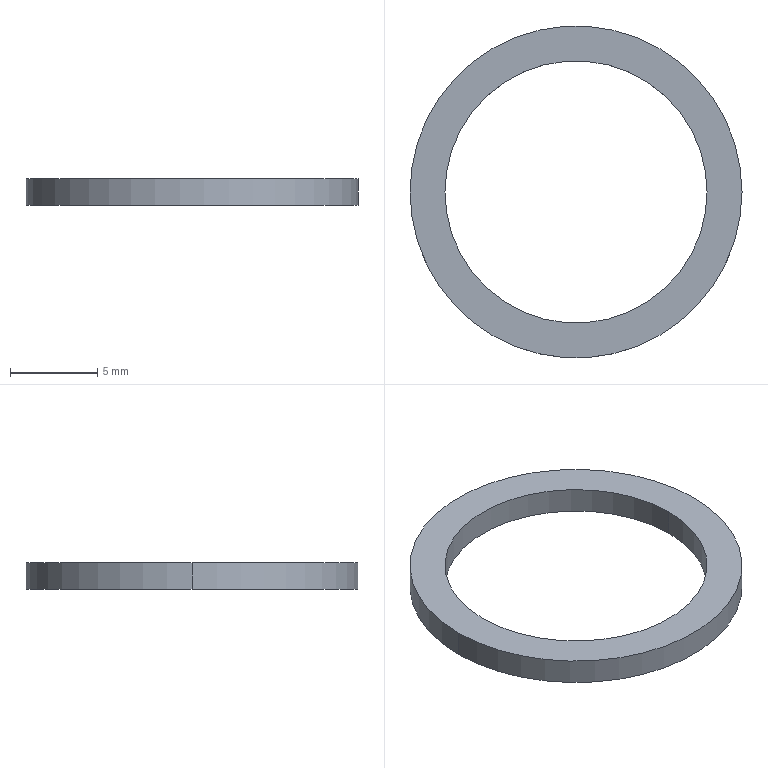Component | SolidWorks | Roller-01-2-1_XT-1-09-2-1 | 1 solid | 6 faces | box 19 x 19 x 1.5 mm | volume 160 mm3 | cylinder 4 | plane 2 | commonest cylinder face diameters 15 x2 19 x2
build123d program:
from build123d import *

# Parameters (mm, degrees)
SKETCH1_R           = 9.5
SKETCH1_R_2         = 7.5
BOSS_EXTRUDE1_DEPTH = 1.5


with BuildPart() as part:
    # Sketch1 → Boss-Extrude1 (new body)
    with BuildSketch(Plane.XY):
        Circle(SKETCH1_R)
        Circle(SKETCH1_R_2, mode=Mode.SUBTRACT)
    extrude(amount=BOSS_EXTRUDE1_DEPTH)


solid = part.part

# Placed as in the assembly
solid = solid.moved(Location((444.783, 71.385, -38), (0, 0, 0)))
STEP:
#1=COLOUR_RGB('',0.7922,0.8196,0.9333);
#2=FILL_AREA_STYLE_COLOUR('',#1);
#3=FILL_AREA_STYLE('',(#2));
#4=SURFACE_STYLE_FILL_AREA(#3);
#5=SURFACE_SIDE_STYLE('',(#4));
#6=SURFACE_STYLE_USAGE(.BOTH.,#5);
#7=PRESENTATION_STYLE_ASSIGNMENT((#6));
#8=CARTESIAN_POINT('',(17.216,2.81,-1.437));
#9=VERTEX_POINT('',#8);
#10=CARTESIAN_POINT('',(17.806,2.81,-1.437));
#11=VERTEX_POINT('',#10);
#12=CARTESIAN_POINT('',(17.511,2.81,-1.437));
#13=DIRECTION('',(0.,0.,1.));
#14=DIRECTION('',(1.,0.,0.));
#15=AXIS2_PLACEMENT_3D('',#12,#13,#14);
#16=CIRCLE('',#15,0.2953);
#17=EDGE_CURVE('',#9,#11,#16,.T.);
#18=ORIENTED_EDGE('',*,*,#17,.T.);
#19=CARTESIAN_POINT('',(17.806,2.81,-1.496));
#20=VERTEX_POINT('',#19);
#21=CARTESIAN_POINT('',(17.806,2.81,-1.437));
#22=DIRECTION('',(0.,0.,-1.));
#23=VECTOR('',#22,39.37);
#24=LINE('',#21,#23);
#25=EDGE_CURVE('',#11,#20,#24,.T.);
#26=ORIENTED_EDGE('',*,*,#25,.T.);
#27=CARTESIAN_POINT('',(17.216,2.81,-1.496));
#28=VERTEX_POINT('',#27);
#29=CARTESIAN_POINT('',(17.511,2.81,-1.496));
#30=DIRECTION('',(0.,0.,1.));
#31=DIRECTION('',(1.,0.,0.));
#32=AXIS2_PLACEMENT_3D('',#29,#30,#31);
#33=CIRCLE('',#32,0.2953);
#34=EDGE_CURVE('',#28,#20,#33,.T.);
#35=ORIENTED_EDGE('',*,*,#34,.F.);
#36=CARTESIAN_POINT('',(17.216,2.81,-1.437));
#37=DIRECTION('',(0.,0.,-1.));
#38=VECTOR('',#37,39.37);
#39=LINE('',#36,#38);
#40=EDGE_CURVE('',#9,#28,#39,.T.);
#41=ORIENTED_EDGE('',*,*,#40,.F.);
#42=EDGE_LOOP('',(#18,#26,#35,#41));
#43=FACE_OUTER_BOUND('',#42,.T.);
#44=CARTESIAN_POINT('',(17.511,2.81,-1.437));
#45=DIRECTION('',(0.,0.,-1.));
#46=DIRECTION('',(-1.,0.,0.));
#47=AXIS2_PLACEMENT_3D('',#44,#45,#46);
#48=CYLINDRICAL_SURFACE('',#47,0.2953);
#49=ADVANCED_FACE('',(#43),#48,.F.);
#50=CARTESIAN_POINT('',(17.885,2.81,-1.437));
#51=VERTEX_POINT('',#50);
#52=CARTESIAN_POINT('',(17.137,2.81,-1.437));
#53=VERTEX_POINT('',#52);
#54=CARTESIAN_POINT('',(17.511,2.81,-1.437));
#55=DIRECTION('',(0.,0.,1.));
#56=DIRECTION('',(1.,0.,0.));
#57=AXIS2_PLACEMENT_3D('',#54,#55,#56);
#58=CIRCLE('',#57,0.374);
#59=EDGE_CURVE('',#51,#53,#58,.T.);
#60=ORIENTED_EDGE('',*,*,#59,.F.);
#61=CARTESIAN_POINT('',(17.885,2.81,-1.496));
#62=VERTEX_POINT('',#61);
#63=CARTESIAN_POINT('',(17.885,2.81,-1.437));
#64=DIRECTION('',(0.,0.,-1.));
#65=VECTOR('',#64,39.37);
#66=LINE('',#63,#65);
#67=EDGE_CURVE('',#51,#62,#66,.T.);
#68=ORIENTED_EDGE('',*,*,#67,.T.);
#69=CARTESIAN_POINT('',(17.137,2.81,-1.496));
#70=VERTEX_POINT('',#69);
#71=CARTESIAN_POINT('',(17.511,2.81,-1.496));
#72=DIRECTION('',(0.,0.,1.));
#73=DIRECTION('',(1.,0.,0.));
#74=AXIS2_PLACEMENT_3D('',#71,#72,#73);
#75=CIRCLE('',#74,0.374);
#76=EDGE_CURVE('',#62,#70,#75,.T.);
#77=ORIENTED_EDGE('',*,*,#76,.T.);
#78=CARTESIAN_POINT('',(17.137,2.81,-1.437));
#79=DIRECTION('',(0.,0.,-1.));
#80=VECTOR('',#79,39.37);
#81=LINE('',#78,#80);
#82=EDGE_CURVE('',#53,#70,#81,.T.);
#83=ORIENTED_EDGE('',*,*,#82,.F.);
#84=EDGE_LOOP('',(#60,#68,#77,#83));
#85=FACE_OUTER_BOUND('',#84,.T.);
#86=CARTESIAN_POINT('',(17.511,2.81,-1.437));
#87=DIRECTION('',(0.,0.,-1.));
#88=DIRECTION('',(-1.,0.,0.));
#89=AXIS2_PLACEMENT_3D('',#86,#87,#88);
#90=CYLINDRICAL_SURFACE('',#89,0.374);
#91=ADVANCED_FACE('',(#85),#90,.T.);
#92=CARTESIAN_POINT('',(17.511,2.81,-1.437));
#93=DIRECTION('',(0.,0.,1.));
#94=DIRECTION('',(1.,0.,0.));
#95=AXIS2_PLACEMENT_3D('',#92,#93,#94);
#96=CIRCLE('',#95,0.374);
#97=EDGE_CURVE('',#53,#51,#96,.T.);
#98=ORIENTED_EDGE('',*,*,#97,.T.);
#99=ORIENTED_EDGE('',*,*,#59,.T.);
#100=EDGE_LOOP('',(#98,#99));
#101=FACE_OUTER_BOUND('',#100,.T.);
#102=ORIENTED_EDGE('',*,*,#17,.F.);
#103=CARTESIAN_POINT('',(17.511,2.81,-1.437));
#104=DIRECTION('',(0.,0.,1.));
#105=DIRECTION('',(1.,0.,0.));
#106=AXIS2_PLACEMENT_3D('',#103,#104,#105);
#107=CIRCLE('',#106,0.2953);
#108=EDGE_CURVE('',#11,#9,#107,.T.);
#109=ORIENTED_EDGE('',*,*,#108,.F.);
#110=EDGE_LOOP('',(#102,#109));
#111=FACE_BOUND('',#110,.T.);
#112=CARTESIAN_POINT('',(17.511,2.81,-1.437));
#113=DIRECTION('',(0.,0.,1.));
#114=DIRECTION('',(1.,0.,0.));
#115=AXIS2_PLACEMENT_3D('',#112,#113,#114);
#116=PLANE('',#115);
#117=ADVANCED_FACE('',(#101,#111),#116,.T.);
#118=CARTESIAN_POINT('',(17.511,2.81,-1.496));
#119=DIRECTION('',(0.,0.,1.));
#120=DIRECTION('',(1.,0.,0.));
#121=AXIS2_PLACEMENT_3D('',#118,#119,#120);
#122=CIRCLE('',#121,0.374);
#123=EDGE_CURVE('',#70,#62,#122,.T.);
#124=ORIENTED_EDGE('',*,*,#123,.F.);
#125=ORIENTED_EDGE('',*,*,#76,.F.);
#126=EDGE_LOOP('',(#124,#125));
#127=FACE_OUTER_BOUND('',#126,.T.);
#128=ORIENTED_EDGE('',*,*,#34,.T.);
#129=CARTESIAN_POINT('',(17.511,2.81,-1.496));
#130=DIRECTION('',(0.,0.,1.));
#131=DIRECTION('',(1.,0.,0.));
#132=AXIS2_PLACEMENT_3D('',#129,#130,#131);
#133=CIRCLE('',#132,0.2953);
#134=EDGE_CURVE('',#20,#28,#133,.T.);
#135=ORIENTED_EDGE('',*,*,#134,.T.);
#136=EDGE_LOOP('',(#128,#135));
#137=FACE_BOUND('',#136,.T.);
#138=CARTESIAN_POINT('',(17.511,2.81,-1.496));
#139=DIRECTION('',(0.,0.,1.));
#140=DIRECTION('',(1.,0.,0.));
#141=AXIS2_PLACEMENT_3D('',#138,#139,#140);
#142=PLANE('',#141);
#143=ADVANCED_FACE('',(#127,#137),#142,.F.);
#144=ORIENTED_EDGE('',*,*,#67,.F.);
#145=ORIENTED_EDGE('',*,*,#97,.F.);
#146=ORIENTED_EDGE('',*,*,#82,.T.);
#147=ORIENTED_EDGE('',*,*,#123,.T.);
#148=EDGE_LOOP('',(#144,#145,#146,#147));
#149=FACE_OUTER_BOUND('',#148,.T.);
#150=CARTESIAN_POINT('',(17.511,2.81,-1.437));
#151=DIRECTION('',(0.,0.,-1.));
#152=DIRECTION('',(-1.,0.,0.));
#153=AXIS2_PLACEMENT_3D('',#150,#151,#152);
#154=CYLINDRICAL_SURFACE('',#153,0.374);
#155=ADVANCED_FACE('',(#149),#154,.T.);
#156=ORIENTED_EDGE('',*,*,#25,.F.);
#157=ORIENTED_EDGE('',*,*,#108,.T.);
#158=ORIENTED_EDGE('',*,*,#40,.T.);
#159=ORIENTED_EDGE('',*,*,#134,.F.);
#160=EDGE_LOOP('',(#156,#157,#158,#159));
#161=FACE_OUTER_BOUND('',#160,.T.);
#162=CARTESIAN_POINT('',(17.511,2.81,-1.437));
#163=DIRECTION('',(0.,0.,-1.));
#164=DIRECTION('',(-1.,0.,0.));
#165=AXIS2_PLACEMENT_3D('',#162,#163,#164);
#166=CYLINDRICAL_SURFACE('',#165,0.2953);
#167=ADVANCED_FACE('',(#161),#166,.F.);
#168=CLOSED_SHELL('',(#49,#91,#117,#143,#155,#167));
#169=MANIFOLD_SOLID_BREP('',#168);
#170=STYLED_ITEM('',(#7),#169);
#171=(LENGTH_UNIT()NAMED_UNIT(*)SI_UNIT($,.METRE.));
#172=LENGTH_MEASURE_WITH_UNIT(LENGTH_MEASURE(0.0254),#171);
#173=DIMENSIONAL_EXPONENTS(1.,0.,0.,0.,0.,0.,0.);
#174=(CONVERSION_BASED_UNIT('',#172)LENGTH_UNIT()NAMED_UNIT(#173));
#175=UNCERTAINTY_MEASURE_WITH_UNIT(LENGTH_MEASURE(0.00001),#174,'','');
#176=(NAMED_UNIT(*)PLANE_ANGLE_UNIT()SI_UNIT($,.RADIAN.));
#177=(NAMED_UNIT(*)SI_UNIT($,.STERADIAN.)SOLID_ANGLE_UNIT());
#178=(GEOMETRIC_REPRESENTATION_CONTEXT(3)GLOBAL_UNCERTAINTY_ASSIGNED_CONTEXT((#175))GLOBAL_UNIT_ASSIGNED_CONTEXT((#174,#176,#177))REPRESENTATION_CONTEXT('',''));
#179=MECHANICAL_DESIGN_GEOMETRIC_PRESENTATION_REPRESENTATION('',(#170),#178);
#180=CARTESIAN_POINT('',(0.,0.,0.));
#181=DIRECTION('',(0.,0.,1.));
#182=DIRECTION('',(1.,0.,0.));
#183=AXIS2_PLACEMENT_3D('',#180,#181,#182);
#184=(LENGTH_UNIT()NAMED_UNIT(*)SI_UNIT($,.METRE.));
#185=LENGTH_MEASURE_WITH_UNIT(LENGTH_MEASURE(0.0254),#184);
#186=DIMENSIONAL_EXPONENTS(1.,0.,0.,0.,0.,0.,0.);
#187=(CONVERSION_BASED_UNIT('',#185)LENGTH_UNIT()NAMED_UNIT(#186));
#188=UNCERTAINTY_MEASURE_WITH_UNIT(LENGTH_MEASURE(0.00001),#187,'','');
#189=(NAMED_UNIT(*)PLANE_ANGLE_UNIT()SI_UNIT($,.RADIAN.));
#190=(NAMED_UNIT(*)SI_UNIT($,.STERADIAN.)SOLID_ANGLE_UNIT());
#191=(GEOMETRIC_REPRESENTATION_CONTEXT(3)GLOBAL_UNCERTAINTY_ASSIGNED_CONTEXT((#188))GLOBAL_UNIT_ASSIGNED_CONTEXT((#187,#189,#190))REPRESENTATION_CONTEXT('',''));
#192=ADVANCED_BREP_SHAPE_REPRESENTATION('',(#169,#183),#191);
#193=PRESENTATION_LAYER_ASSIGNMENT('','',(#170));